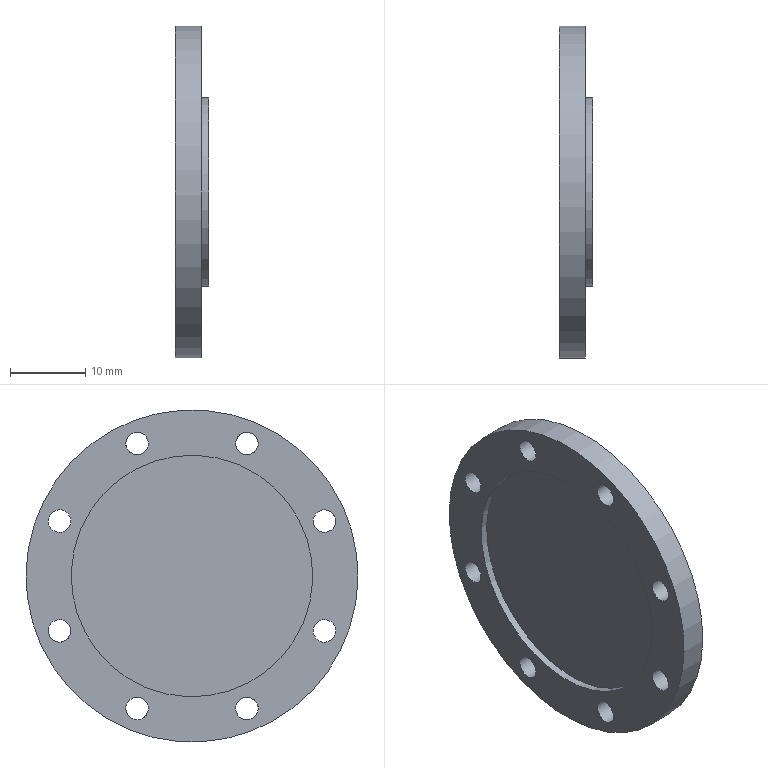Component | NX | END_COVER_1 | 1 solid | 15 faces | volume 4811 mm3 | cylinder 11 | plane 4 | commonest cylinder face diameters 3 x8 25 x1 44 x1 32 x1